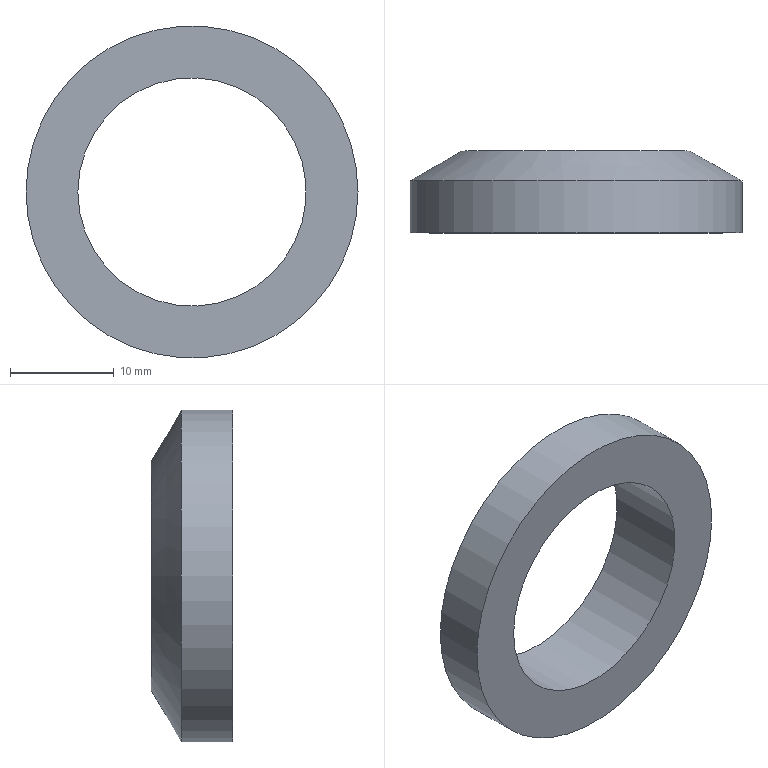Component | NX | PACKING | 1 solid | 4 faces | box 32 x 7.89 x 32 mm | volume 2695 mm3 | cylinder 2 | plane 1 | cone 1 | commonest cylinder face diameters 32 x1 22 x1
STEP:
#1=CARTESIAN_POINT('',(0.,0.,0.));
#2=DIRECTION('',(0.,0.,1.));
#3=DIRECTION('',(1.,0.,0.));
#4=AXIS2_PLACEMENT_3D('',#1,#2,#3);
#5=CARTESIAN_POINT('',(-16.,19.5,10.75));
#6=VERTEX_POINT('',#5);
#7=CARTESIAN_POINT('',(-0.,19.5,10.75));
#8=DIRECTION('',(0.,-1.,0.));
#9=DIRECTION('',(-1.,0.,0.));
#10=AXIS2_PLACEMENT_3D('',#7,#8,#9);
#11=CIRCLE('',#10,16.);
#12=CARTESIAN_POINT('',(-0.,19.5,21.75));
#13=DIRECTION('',(0.,-1.,0.));
#14=DIRECTION('',(-1.,0.,0.));
#15=AXIS2_PLACEMENT_3D('',#12,#13,#14);
#16=PLANE('',#15);
#17=CARTESIAN_POINT('',(0.,11.));
#18=DIRECTION('',(1.,0.));
#19=AXIS2_PLACEMENT_2D('',#17,#18);
#20=CIRCLE('',#19,16.);
#21=(GEOMETRIC_REPRESENTATION_CONTEXT(2)PARAMETRIC_REPRESENTATION_CONTEXT()REPRESENTATION_CONTEXT('',''));
#22=DEFINITIONAL_REPRESENTATION('',(#20),#21);
#23=PCURVE('',#16,#22);
#24=CARTESIAN_POINT('',(-0.,19.5,10.75));
#25=DIRECTION('',(0.,-1.,0.));
#26=DIRECTION('',(-1.,0.,0.));
#27=AXIS2_PLACEMENT_3D('',#24,#25,#26);
#28=CYLINDRICAL_SURFACE('',#27,16.);
#29=CARTESIAN_POINT('',(0.,0.));
#30=DIRECTION('',(1.,0.));
#31=VECTOR('',#30,1.);
#32=LINE('',#29,#31);
#33=(GEOMETRIC_REPRESENTATION_CONTEXT(2)PARAMETRIC_REPRESENTATION_CONTEXT()REPRESENTATION_CONTEXT('',''));
#34=DEFINITIONAL_REPRESENTATION('',(#32),#33);
#35=PCURVE('',#28,#34);
#36=SURFACE_CURVE('',#11,(#23,#35),.PCURVE_S1.);
#37=EDGE_CURVE('',#6,#6,#36,.T.);
#38=ORIENTED_EDGE('',*,*,#37,.T.);
#39=EDGE_LOOP('',(#38));
#40=FACE_BOUND('',#39,.T.);
#41=CARTESIAN_POINT('',(-11.,19.5,10.75));
#42=VERTEX_POINT('',#41);
#43=CARTESIAN_POINT('',(-0.,19.5,10.75));
#44=DIRECTION('',(0.,-1.,0.));
#45=DIRECTION('',(-1.,0.,0.));
#46=AXIS2_PLACEMENT_3D('',#43,#44,#45);
#47=CIRCLE('',#46,11.);
#48=CARTESIAN_POINT('',(0.,11.));
#49=DIRECTION('',(1.,0.));
#50=AXIS2_PLACEMENT_2D('',#48,#49);
#51=CIRCLE('',#50,11.);
#52=(GEOMETRIC_REPRESENTATION_CONTEXT(2)PARAMETRIC_REPRESENTATION_CONTEXT()REPRESENTATION_CONTEXT('',''));
#53=DEFINITIONAL_REPRESENTATION('',(#51),#52);
#54=PCURVE('',#16,#53);
#55=CARTESIAN_POINT('',(-0.,19.5,10.75));
#56=DIRECTION('',(0.,-1.,0.));
#57=DIRECTION('',(-1.,0.,0.));
#58=AXIS2_PLACEMENT_3D('',#55,#56,#57);
#59=CYLINDRICAL_SURFACE('',#58,11.);
#60=CARTESIAN_POINT('',(0.,0.));
#61=DIRECTION('',(1.,0.));
#62=VECTOR('',#61,1.);
#63=LINE('',#60,#62);
#64=(GEOMETRIC_REPRESENTATION_CONTEXT(2)PARAMETRIC_REPRESENTATION_CONTEXT()REPRESENTATION_CONTEXT('',''));
#65=DEFINITIONAL_REPRESENTATION('',(#63),#64);
#66=PCURVE('',#59,#65);
#67=SURFACE_CURVE('',#47,(#54,#66),.PCURVE_S1.);
#68=EDGE_CURVE('',#42,#42,#67,.T.);
#69=ORIENTED_EDGE('',*,*,#68,.F.);
#70=EDGE_LOOP('',(#69));
#71=FACE_BOUND('',#70,.T.);
#72=ADVANCED_FACE('',(#40,#71),#16,.T.);
#73=CARTESIAN_POINT('',(-16.,24.5,10.75));
#74=VERTEX_POINT('',#73);
#75=CARTESIAN_POINT('',(-0.,24.5,10.75));
#76=DIRECTION('',(0.,-1.,0.));
#77=DIRECTION('',(-1.,0.,0.));
#78=AXIS2_PLACEMENT_3D('',#75,#76,#77);
#79=CIRCLE('',#78,16.);
#80=CARTESIAN_POINT('',(0.,-5.));
#81=DIRECTION('',(1.,0.));
#82=VECTOR('',#81,1.);
#83=LINE('',#80,#82);
#84=(GEOMETRIC_REPRESENTATION_CONTEXT(2)PARAMETRIC_REPRESENTATION_CONTEXT()REPRESENTATION_CONTEXT('',''));
#85=DEFINITIONAL_REPRESENTATION('',(#83),#84);
#86=PCURVE('',#28,#85);
#87=CARTESIAN_POINT('',(-0.,24.5,10.75));
#88=DIRECTION('',(0.,-1.,0.));
#89=DIRECTION('',(-1.,0.,0.));
#90=AXIS2_PLACEMENT_3D('',#87,#88,#89);
#91=CONICAL_SURFACE('',#90,16.,1.047);
#92=CARTESIAN_POINT('',(0.,0.));
#93=DIRECTION('',(1.,0.));
#94=VECTOR('',#93,1.);
#95=LINE('',#92,#94);
#96=(GEOMETRIC_REPRESENTATION_CONTEXT(2)PARAMETRIC_REPRESENTATION_CONTEXT()REPRESENTATION_CONTEXT('',''));
#97=DEFINITIONAL_REPRESENTATION('',(#95),#96);
#98=PCURVE('',#91,#97);
#99=SURFACE_CURVE('',#79,(#86,#98),.PCURVE_S1.);
#100=EDGE_CURVE('',#74,#74,#99,.T.);
#101=ORIENTED_EDGE('',*,*,#100,.T.);
#102=CARTESIAN_POINT('',(-16.,24.5,10.75));
#103=CARTESIAN_POINT('',(-16.,19.5,10.75));
#104=B_SPLINE_CURVE_WITH_KNOTS('',1,(#102,#103),.UNSPECIFIED.,.F.,.F.,(2,2),(-5.,0.),.PIECEWISE_BEZIER_KNOTS.);
#105=CARTESIAN_POINT('',(6.283,0.));
#106=DIRECTION('',(0.,1.));
#107=VECTOR('',#106,1.);
#108=LINE('',#105,#107);
#109=(GEOMETRIC_REPRESENTATION_CONTEXT(2)PARAMETRIC_REPRESENTATION_CONTEXT()REPRESENTATION_CONTEXT('',''));
#110=DEFINITIONAL_REPRESENTATION('',(#108),#109);
#111=PCURVE('',#28,#110);
#112=CARTESIAN_POINT('',(0.,0.));
#113=DIRECTION('',(0.,1.));
#114=VECTOR('',#113,1.);
#115=LINE('',#112,#114);
#116=(GEOMETRIC_REPRESENTATION_CONTEXT(2)PARAMETRIC_REPRESENTATION_CONTEXT()REPRESENTATION_CONTEXT('',''));
#117=DEFINITIONAL_REPRESENTATION('',(#115),#116);
#118=PCURVE('',#28,#117);
#119=SEAM_CURVE('',#104,(#111,#118),.PCURVE_S1.);
#120=EDGE_CURVE('',#74,#6,#119,.T.);
#121=ORIENTED_EDGE('',*,*,#120,.T.);
#122=ORIENTED_EDGE('',*,*,#37,.F.);
#123=ORIENTED_EDGE('',*,*,#120,.F.);
#124=EDGE_LOOP('',(#101,#121,#122,#123));
#125=FACE_BOUND('',#124,.T.);
#126=ADVANCED_FACE('',(#125),#28,.T.);
#127=CARTESIAN_POINT('',(-11.,27.387,10.75));
#128=VERTEX_POINT('',#127);
#129=CARTESIAN_POINT('',(-0.,27.387,10.75));
#130=DIRECTION('',(0.,-1.,0.));
#131=DIRECTION('',(-1.,0.,0.));
#132=AXIS2_PLACEMENT_3D('',#129,#130,#131);
#133=CIRCLE('',#132,11.);
#134=CARTESIAN_POINT('',(0.,-2.887));
#135=DIRECTION('',(1.,0.));
#136=VECTOR('',#135,1.);
#137=LINE('',#134,#136);
#138=(GEOMETRIC_REPRESENTATION_CONTEXT(2)PARAMETRIC_REPRESENTATION_CONTEXT()REPRESENTATION_CONTEXT('',''));
#139=DEFINITIONAL_REPRESENTATION('',(#137),#138);
#140=PCURVE('',#91,#139);
#141=CARTESIAN_POINT('',(0.,-7.887));
#142=DIRECTION('',(1.,0.));
#143=VECTOR('',#142,1.);
#144=LINE('',#141,#143);
#145=(GEOMETRIC_REPRESENTATION_CONTEXT(2)PARAMETRIC_REPRESENTATION_CONTEXT()REPRESENTATION_CONTEXT('',''));
#146=DEFINITIONAL_REPRESENTATION('',(#144),#145);
#147=PCURVE('',#59,#146);
#148=SURFACE_CURVE('',#133,(#140,#147),.PCURVE_S1.);
#149=EDGE_CURVE('',#128,#128,#148,.T.);
#150=ORIENTED_EDGE('',*,*,#149,.T.);
#151=CARTESIAN_POINT('',(-11.,27.387,10.75));
#152=CARTESIAN_POINT('',(-16.,24.5,10.75));
#153=B_SPLINE_CURVE_WITH_KNOTS('',1,(#151,#152),.UNSPECIFIED.,.F.,.F.,(2,2),(-5.774,0.),.PIECEWISE_BEZIER_KNOTS.);
#154=CARTESIAN_POINT('',(6.283,0.));
#155=DIRECTION('',(0.,1.));
#156=VECTOR('',#155,1.);
#157=LINE('',#154,#156);
#158=(GEOMETRIC_REPRESENTATION_CONTEXT(2)PARAMETRIC_REPRESENTATION_CONTEXT()REPRESENTATION_CONTEXT('',''));
#159=DEFINITIONAL_REPRESENTATION('',(#157),#158);
#160=PCURVE('',#91,#159);
#161=CARTESIAN_POINT('',(0.,0.));
#162=DIRECTION('',(0.,1.));
#163=VECTOR('',#162,1.);
#164=LINE('',#161,#163);
#165=(GEOMETRIC_REPRESENTATION_CONTEXT(2)PARAMETRIC_REPRESENTATION_CONTEXT()REPRESENTATION_CONTEXT('',''));
#166=DEFINITIONAL_REPRESENTATION('',(#164),#165);
#167=PCURVE('',#91,#166);
#168=SEAM_CURVE('',#153,(#160,#167),.PCURVE_S1.);
#169=EDGE_CURVE('',#128,#74,#168,.T.);
#170=ORIENTED_EDGE('',*,*,#169,.T.);
#171=ORIENTED_EDGE('',*,*,#100,.F.);
#172=ORIENTED_EDGE('',*,*,#169,.F.);
#173=EDGE_LOOP('',(#150,#170,#171,#172));
#174=FACE_BOUND('',#173,.T.);
#175=ADVANCED_FACE('',(#174),#91,.T.);
#176=ORIENTED_EDGE('',*,*,#68,.F.);
#177=CARTESIAN_POINT('',(-11.,27.387,10.75));
#178=CARTESIAN_POINT('',(-11.,19.5,10.75));
#179=B_SPLINE_CURVE_WITH_KNOTS('',1,(#177,#178),.UNSPECIFIED.,.F.,.F.,(2,2),(-7.887,0.),.PIECEWISE_BEZIER_KNOTS.);
#180=CARTESIAN_POINT('',(0.,0.));
#181=DIRECTION('',(0.,1.));
#182=VECTOR('',#181,1.);
#183=LINE('',#180,#182);
#184=(GEOMETRIC_REPRESENTATION_CONTEXT(2)PARAMETRIC_REPRESENTATION_CONTEXT()REPRESENTATION_CONTEXT('',''));
#185=DEFINITIONAL_REPRESENTATION('',(#183),#184);
#186=PCURVE('',#59,#185);
#187=CARTESIAN_POINT('',(6.283,0.));
#188=DIRECTION('',(0.,1.));
#189=VECTOR('',#188,1.);
#190=LINE('',#187,#189);
#191=(GEOMETRIC_REPRESENTATION_CONTEXT(2)PARAMETRIC_REPRESENTATION_CONTEXT()REPRESENTATION_CONTEXT('',''));
#192=DEFINITIONAL_REPRESENTATION('',(#190),#191);
#193=PCURVE('',#59,#192);
#194=SEAM_CURVE('',#179,(#186,#193),.PCURVE_S1.);
#195=EDGE_CURVE('',#128,#42,#194,.T.);
#196=ORIENTED_EDGE('',*,*,#195,.F.);
#197=ORIENTED_EDGE('',*,*,#149,.T.);
#198=ORIENTED_EDGE('',*,*,#195,.T.);
#199=EDGE_LOOP('',(#176,#196,#197,#198));
#200=FACE_BOUND('',#199,.F.);
#201=ADVANCED_FACE('',(#200),#59,.F.);
#202=CLOSED_SHELL('',(#72,#126,#175,#201));
#203=MANIFOLD_SOLID_BREP('',#202);
#204=(LENGTH_UNIT()NAMED_UNIT(*)SI_UNIT(.MILLI.,.METRE.));
#205=UNCERTAINTY_MEASURE_WITH_UNIT(LENGTH_MEASURE(0.00001),#204,'','');
#206=(NAMED_UNIT(*)PLANE_ANGLE_UNIT()SI_UNIT($,.RADIAN.));
#207=(NAMED_UNIT(*)SI_UNIT($,.STERADIAN.)SOLID_ANGLE_UNIT());
#208=(GEOMETRIC_REPRESENTATION_CONTEXT(3)GLOBAL_UNCERTAINTY_ASSIGNED_CONTEXT((#205))GLOBAL_UNIT_ASSIGNED_CONTEXT((#204,#206,#207))REPRESENTATION_CONTEXT('',''));
#209=ADVANCED_BREP_SHAPE_REPRESENTATION('',(#4,#203),#208);